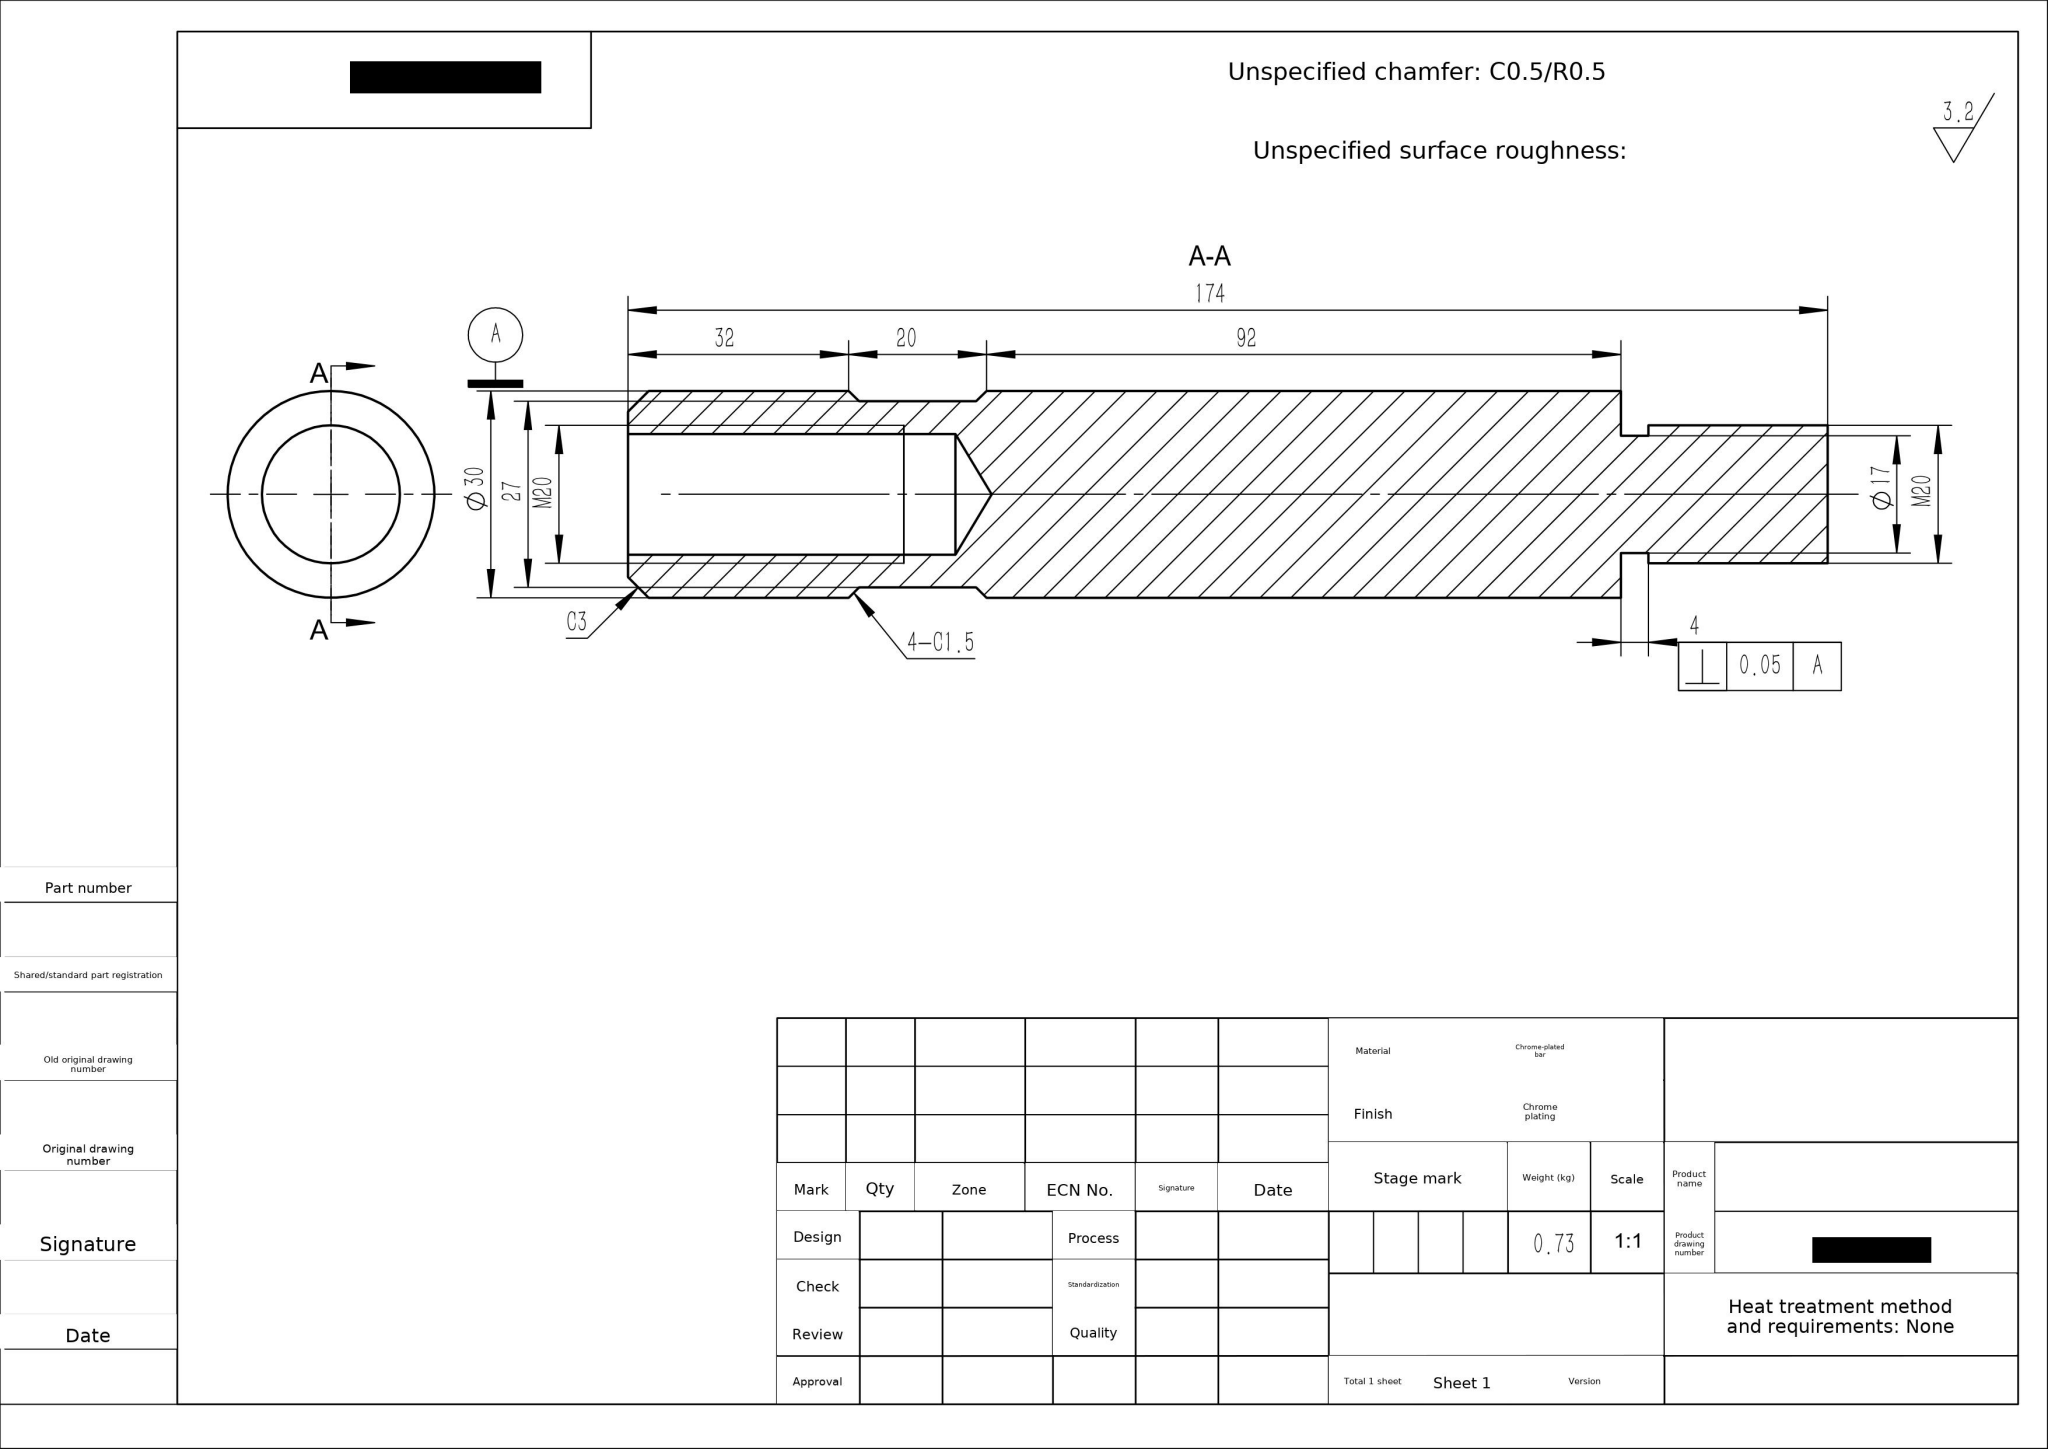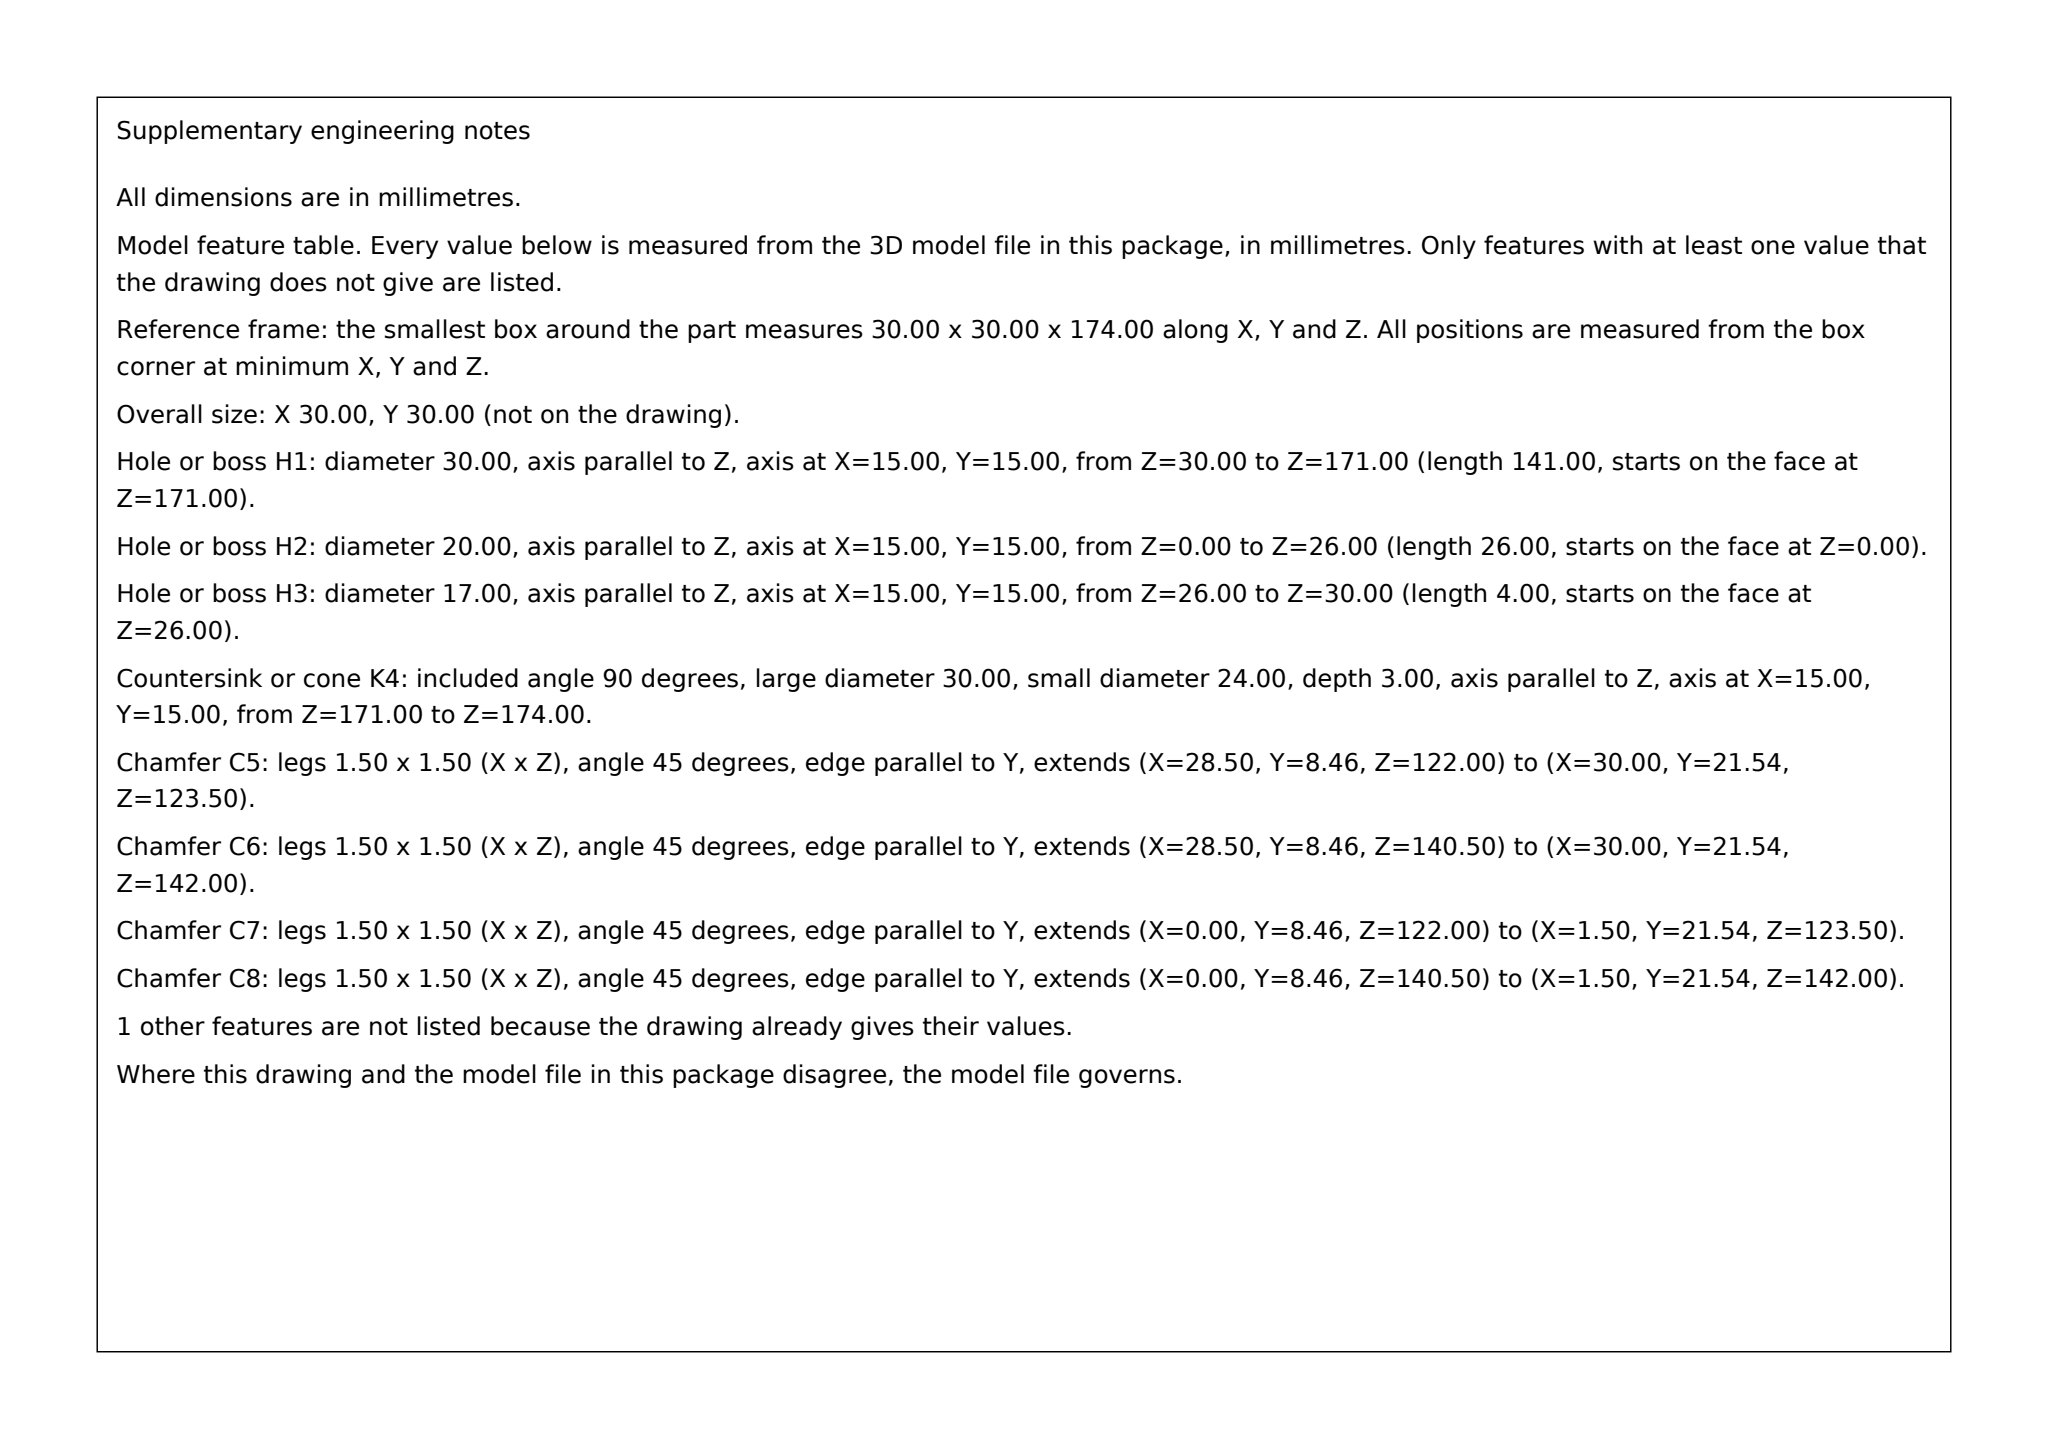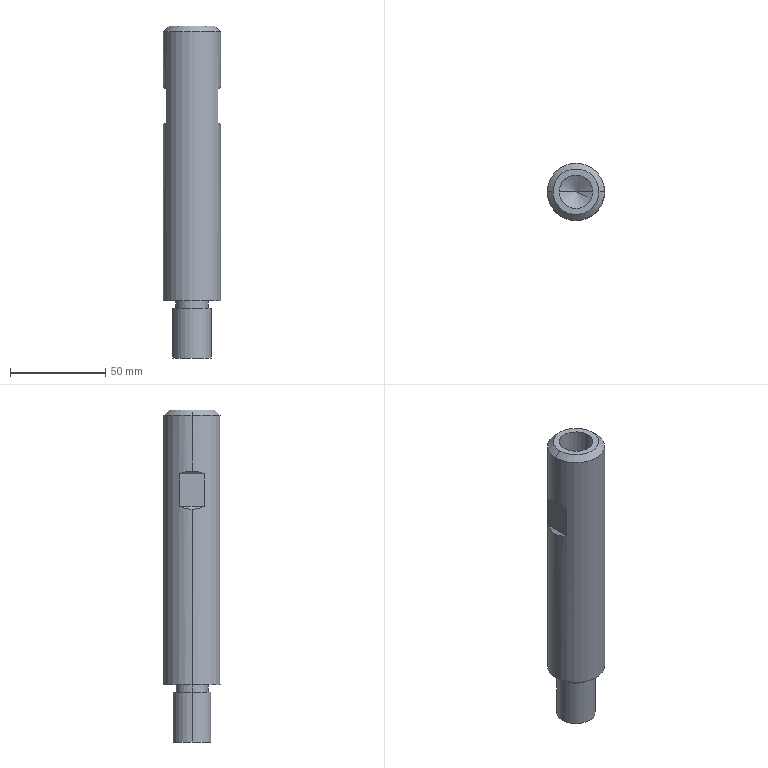Part | SolidWorks | mm | material Chrome-plated bar | 1 solid | 22 faces | box 30 x 30 x 174 mm | volume 98140 mm3 | plane 10 | cylinder 8 | cone 4 | commonest cylinder face diameters 20 x2 17 x2 17.5 x2 30 x2
STEP:
#1=CARTESIAN_POINT('',(12.,0.,174.));
#2=VERTEX_POINT('',#1);
#3=CARTESIAN_POINT('',(-12.,0.,174.));
#4=VERTEX_POINT('',#3);
#5=CARTESIAN_POINT('',(0.,0.,174.));
#6=DIRECTION('',(0.,0.,1.));
#7=DIRECTION('',(1.,0.,0.));
#8=AXIS2_PLACEMENT_3D('',#5,#6,#7);
#9=CIRCLE('',#8,12.);
#10=EDGE_CURVE('',#2,#4,#9,.T.);
#11=ORIENTED_EDGE('',*,*,#10,.F.);
#12=CARTESIAN_POINT('',(15.,0.,171.));
#13=VERTEX_POINT('',#12);
#14=CARTESIAN_POINT('',(12.,0.,174.));
#15=DIRECTION('',(0.7071,0.,-0.7071));
#16=VECTOR('',#15,1000.);
#17=LINE('',#14,#16);
#18=EDGE_CURVE('',#2,#13,#17,.T.);
#19=ORIENTED_EDGE('',*,*,#18,.T.);
#20=CARTESIAN_POINT('',(-15.,0.,171.));
#21=VERTEX_POINT('',#20);
#22=CARTESIAN_POINT('',(0.,0.,171.));
#23=DIRECTION('',(0.,0.,-1.));
#24=DIRECTION('',(1.,0.,0.));
#25=AXIS2_PLACEMENT_3D('',#22,#23,#24);
#26=CIRCLE('',#25,15.);
#27=EDGE_CURVE('',#21,#13,#26,.T.);
#28=ORIENTED_EDGE('',*,*,#27,.F.);
#29=CARTESIAN_POINT('',(-12.,0.,174.));
#30=DIRECTION('',(-0.7071,0.,-0.7071));
#31=VECTOR('',#30,1000.);
#32=LINE('',#29,#31);
#33=EDGE_CURVE('',#4,#21,#32,.T.);
#34=ORIENTED_EDGE('',*,*,#33,.F.);
#35=EDGE_LOOP('',(#11,#19,#28,#34));
#36=FACE_OUTER_BOUND('',#35,.T.);
#37=CARTESIAN_POINT('',(0.,0.,174.));
#38=DIRECTION('',(0.,0.,-1.));
#39=DIRECTION('',(-1.,0.,0.));
#40=AXIS2_PLACEMENT_3D('',#37,#38,#39);
#41=CONICAL_SURFACE('',#40,12.,0.7854);
#42=ADVANCED_FACE('',(#36),#41,.T.);
#43=CARTESIAN_POINT('',(10.,0.,26.));
#44=VERTEX_POINT('',#43);
#45=CARTESIAN_POINT('',(-10.,0.,26.));
#46=VERTEX_POINT('',#45);
#47=CARTESIAN_POINT('',(0.,0.,26.));
#48=DIRECTION('',(0.,0.,1.));
#49=DIRECTION('',(-1.,0.,0.));
#50=AXIS2_PLACEMENT_3D('',#47,#48,#49);
#51=CIRCLE('',#50,10.);
#52=EDGE_CURVE('',#44,#46,#51,.T.);
#53=ORIENTED_EDGE('',*,*,#52,.F.);
#54=CARTESIAN_POINT('',(10.,0.,0.));
#55=VERTEX_POINT('',#54);
#56=CARTESIAN_POINT('',(10.,0.,30.));
#57=DIRECTION('',(0.,0.,-1.));
#58=VECTOR('',#57,1000.);
#59=LINE('',#56,#58);
#60=EDGE_CURVE('',#44,#55,#59,.T.);
#61=ORIENTED_EDGE('',*,*,#60,.T.);
#62=CARTESIAN_POINT('',(-10.,0.,0.));
#63=VERTEX_POINT('',#62);
#64=CARTESIAN_POINT('',(0.,0.,0.));
#65=DIRECTION('',(0.,0.,-1.));
#66=DIRECTION('',(-1.,0.,0.));
#67=AXIS2_PLACEMENT_3D('',#64,#65,#66);
#68=CIRCLE('',#67,10.);
#69=EDGE_CURVE('',#63,#55,#68,.T.);
#70=ORIENTED_EDGE('',*,*,#69,.F.);
#71=CARTESIAN_POINT('',(-10.,0.,30.));
#72=DIRECTION('',(0.,0.,-1.));
#73=VECTOR('',#72,1000.);
#74=LINE('',#71,#73);
#75=EDGE_CURVE('',#46,#63,#74,.T.);
#76=ORIENTED_EDGE('',*,*,#75,.F.);
#77=EDGE_LOOP('',(#53,#61,#70,#76));
#78=FACE_OUTER_BOUND('',#77,.T.);
#79=CARTESIAN_POINT('',(0.,0.,30.));
#80=DIRECTION('',(0.,0.,-1.));
#81=DIRECTION('',(-1.,0.,0.));
#82=AXIS2_PLACEMENT_3D('',#79,#80,#81);
#83=CYLINDRICAL_SURFACE('',#82,10.);
#84=ADVANCED_FACE('',(#78),#83,.T.);
#85=CARTESIAN_POINT('',(-8.5,0.,26.));
#86=VERTEX_POINT('',#85);
#87=CARTESIAN_POINT('',(8.5,0.,26.));
#88=VERTEX_POINT('',#87);
#89=CARTESIAN_POINT('',(0.,0.,26.));
#90=DIRECTION('',(0.,0.,-1.));
#91=DIRECTION('',(-1.,0.,0.));
#92=AXIS2_PLACEMENT_3D('',#89,#90,#91);
#93=CIRCLE('',#92,8.5);
#94=EDGE_CURVE('',#86,#88,#93,.T.);
#95=ORIENTED_EDGE('',*,*,#94,.F.);
#96=CARTESIAN_POINT('',(-8.5,0.,30.));
#97=VERTEX_POINT('',#96);
#98=CARTESIAN_POINT('',(-8.5,0.,26.));
#99=DIRECTION('',(0.,0.,1.));
#100=VECTOR('',#99,1000.);
#101=LINE('',#98,#100);
#102=EDGE_CURVE('',#86,#97,#101,.T.);
#103=ORIENTED_EDGE('',*,*,#102,.T.);
#104=CARTESIAN_POINT('',(8.5,0.,30.));
#105=VERTEX_POINT('',#104);
#106=CARTESIAN_POINT('',(0.,0.,30.));
#107=DIRECTION('',(0.,0.,-1.));
#108=DIRECTION('',(-1.,0.,0.));
#109=AXIS2_PLACEMENT_3D('',#106,#107,#108);
#110=CIRCLE('',#109,8.5);
#111=EDGE_CURVE('',#97,#105,#110,.T.);
#112=ORIENTED_EDGE('',*,*,#111,.T.);
#113=CARTESIAN_POINT('',(8.5,0.,26.));
#114=DIRECTION('',(0.,0.,1.));
#115=VECTOR('',#114,1000.);
#116=LINE('',#113,#115);
#117=EDGE_CURVE('',#88,#105,#116,.T.);
#118=ORIENTED_EDGE('',*,*,#117,.F.);
#119=EDGE_LOOP('',(#95,#103,#112,#118));
#120=FACE_OUTER_BOUND('',#119,.T.);
#121=CARTESIAN_POINT('',(0.,0.,26.));
#122=DIRECTION('',(0.,0.,1.));
#123=DIRECTION('',(1.,0.,0.));
#124=AXIS2_PLACEMENT_3D('',#121,#122,#123);
#125=CYLINDRICAL_SURFACE('',#124,8.5);
#126=ADVANCED_FACE('',(#120),#125,.T.);
#127=CARTESIAN_POINT('',(-8.75,0.,126.5));
#128=VERTEX_POINT('',#127);
#129=CARTESIAN_POINT('',(8.75,0.,126.5));
#130=VERTEX_POINT('',#129);
#131=CARTESIAN_POINT('',(0.,0.,126.5));
#132=DIRECTION('',(0.,0.,1.));
#133=DIRECTION('',(1.,0.,0.));
#134=AXIS2_PLACEMENT_3D('',#131,#132,#133);
#135=CIRCLE('',#134,8.75);
#136=EDGE_CURVE('',#128,#130,#135,.T.);
#137=ORIENTED_EDGE('',*,*,#136,.F.);
#138=CARTESIAN_POINT('',(-8.75,0.,174.));
#139=VERTEX_POINT('',#138);
#140=CARTESIAN_POINT('',(-8.75,0.,174.));
#141=DIRECTION('',(0.,0.,1.));
#142=VECTOR('',#141,1000.);
#143=LINE('',#140,#142);
#144=EDGE_CURVE('',#128,#139,#143,.T.);
#145=ORIENTED_EDGE('',*,*,#144,.T.);
#146=CARTESIAN_POINT('',(8.75,0.,174.));
#147=VERTEX_POINT('',#146);
#148=CARTESIAN_POINT('',(0.,0.,174.));
#149=DIRECTION('',(0.,0.,1.));
#150=DIRECTION('',(1.,0.,0.));
#151=AXIS2_PLACEMENT_3D('',#148,#149,#150);
#152=CIRCLE('',#151,8.75);
#153=EDGE_CURVE('',#139,#147,#152,.T.);
#154=ORIENTED_EDGE('',*,*,#153,.T.);
#155=CARTESIAN_POINT('',(8.75,0.,174.));
#156=DIRECTION('',(0.,0.,1.));
#157=VECTOR('',#156,1000.);
#158=LINE('',#155,#157);
#159=EDGE_CURVE('',#130,#147,#158,.T.);
#160=ORIENTED_EDGE('',*,*,#159,.F.);
#161=EDGE_LOOP('',(#137,#145,#154,#160));
#162=FACE_OUTER_BOUND('',#161,.T.);
#163=CARTESIAN_POINT('',(0.,0.,174.));
#164=DIRECTION('',(0.,0.,1.));
#165=DIRECTION('',(1.,0.,0.));
#166=AXIS2_PLACEMENT_3D('',#163,#164,#165);
#167=CYLINDRICAL_SURFACE('',#166,8.75);
#168=ADVANCED_FACE('',(#162),#167,.F.);
#169=CARTESIAN_POINT('',(-0.,0.,121.242));
#170=VERTEX_POINT('',#169);
#171=CARTESIAN_POINT('',(8.75,0.,126.5));
#172=DIRECTION('',(0.8572,0.,0.515));
#173=VECTOR('',#172,1000.);
#174=LINE('',#171,#173);
#175=EDGE_CURVE('',#170,#130,#174,.T.);
#176=ORIENTED_EDGE('',*,*,#175,.F.);
#177=CARTESIAN_POINT('',(-8.75,0.,126.5));
#178=DIRECTION('',(-0.8572,0.,0.515));
#179=VECTOR('',#178,1000.);
#180=LINE('',#177,#179);
#181=EDGE_CURVE('',#170,#128,#180,.T.);
#182=ORIENTED_EDGE('',*,*,#181,.T.);
#183=ORIENTED_EDGE('',*,*,#136,.T.);
#184=EDGE_LOOP('',(#176,#182,#183));
#185=FACE_OUTER_BOUND('',#184,.T.);
#186=CARTESIAN_POINT('',(0.,0.,126.5));
#187=DIRECTION('',(0.,0.,1.));
#188=DIRECTION('',(1.,0.,0.));
#189=AXIS2_PLACEMENT_3D('',#186,#187,#188);
#190=CONICAL_SURFACE('',#189,8.75,1.03);
#191=ADVANCED_FACE('',(#185),#190,.F.);
#192=ORIENTED_EDGE('',*,*,#27,.T.);
#193=CARTESIAN_POINT('',(15.,0.,142.));
#194=VERTEX_POINT('',#193);
#195=CARTESIAN_POINT('',(15.,0.,174.));
#196=DIRECTION('',(0.,0.,-1.));
#197=VECTOR('',#196,1000.);
#198=LINE('',#195,#197);
#199=EDGE_CURVE('',#13,#194,#198,.T.);
#200=ORIENTED_EDGE('',*,*,#199,.T.);
#201=CARTESIAN_POINT('',(13.5,6.538,140.5));
#202=VERTEX_POINT('',#201);
#203=CARTESIAN_POINT('',(15.,0.,142.));
#204=CARTESIAN_POINT('',(15.,2.274,142.));
#205=CARTESIAN_POINT('',(14.491,4.491,141.491));
#206=CARTESIAN_POINT('',(13.5,6.538,140.5));
#207=(BOUNDED_CURVE()B_SPLINE_CURVE(3,(#203,#204,#205,#206),.UNSPECIFIED.,.F.,.T.)B_SPLINE_CURVE_WITH_KNOTS((4,4),(3.142,3.593),.UNSPECIFIED.)CURVE()GEOMETRIC_REPRESENTATION_ITEM()RATIONAL_B_SPLINE_CURVE((1.,0.9831,0.9831,1.))REPRESENTATION_ITEM(''));
#208=EDGE_CURVE('',#194,#202,#207,.T.);
#209=ORIENTED_EDGE('',*,*,#208,.T.);
#210=CARTESIAN_POINT('',(13.5,6.538,123.5));
#211=VERTEX_POINT('',#210);
#212=CARTESIAN_POINT('',(13.5,6.538,174.));
#213=DIRECTION('',(0.,0.,1.));
#214=VECTOR('',#213,1000.);
#215=LINE('',#212,#214);
#216=EDGE_CURVE('',#211,#202,#215,.T.);
#217=ORIENTED_EDGE('',*,*,#216,.F.);
#218=CARTESIAN_POINT('',(15.,0.,122.));
#219=VERTEX_POINT('',#218);
#220=CARTESIAN_POINT('',(13.5,6.538,123.5));
#221=CARTESIAN_POINT('',(14.491,4.491,122.509));
#222=CARTESIAN_POINT('',(15.,2.274,122.));
#223=CARTESIAN_POINT('',(15.,0.,122.));
#224=(BOUNDED_CURVE()B_SPLINE_CURVE(3,(#220,#221,#222,#223),.UNSPECIFIED.,.F.,.T.)B_SPLINE_CURVE_WITH_KNOTS((4,4),(5.832,6.283),.UNSPECIFIED.)CURVE()GEOMETRIC_REPRESENTATION_ITEM()RATIONAL_B_SPLINE_CURVE((1.,0.9831,0.9831,1.))REPRESENTATION_ITEM(''));
#225=EDGE_CURVE('',#211,#219,#224,.T.);
#226=ORIENTED_EDGE('',*,*,#225,.T.);
#227=CARTESIAN_POINT('',(15.,0.,30.));
#228=VERTEX_POINT('',#227);
#229=CARTESIAN_POINT('',(15.,0.,174.));
#230=DIRECTION('',(0.,0.,-1.));
#231=VECTOR('',#230,1000.);
#232=LINE('',#229,#231);
#233=EDGE_CURVE('',#219,#228,#232,.T.);
#234=ORIENTED_EDGE('',*,*,#233,.T.);
#235=CARTESIAN_POINT('',(-15.,0.,30.));
#236=VERTEX_POINT('',#235);
#237=CARTESIAN_POINT('',(0.,0.,30.));
#238=DIRECTION('',(0.,0.,-1.));
#239=DIRECTION('',(-1.,0.,0.));
#240=AXIS2_PLACEMENT_3D('',#237,#238,#239);
#241=CIRCLE('',#240,15.);
#242=EDGE_CURVE('',#236,#228,#241,.T.);
#243=ORIENTED_EDGE('',*,*,#242,.F.);
#244=CARTESIAN_POINT('',(-15.,0.,122.));
#245=VERTEX_POINT('',#244);
#246=CARTESIAN_POINT('',(-15.,0.,174.));
#247=DIRECTION('',(0.,0.,-1.));
#248=VECTOR('',#247,1000.);
#249=LINE('',#246,#248);
#250=EDGE_CURVE('',#245,#236,#249,.T.);
#251=ORIENTED_EDGE('',*,*,#250,.F.);
#252=CARTESIAN_POINT('',(-13.5,6.538,123.5));
#253=VERTEX_POINT('',#252);
#254=CARTESIAN_POINT('',(-15.,0.,122.));
#255=CARTESIAN_POINT('',(-15.,2.274,122.));
#256=CARTESIAN_POINT('',(-14.491,4.491,122.509));
#257=CARTESIAN_POINT('',(-13.5,6.538,123.5));
#258=(BOUNDED_CURVE()B_SPLINE_CURVE(3,(#254,#255,#256,#257),.UNSPECIFIED.,.F.,.T.)B_SPLINE_CURVE_WITH_KNOTS((4,4),(0.,0.451),.UNSPECIFIED.)CURVE()GEOMETRIC_REPRESENTATION_ITEM()RATIONAL_B_SPLINE_CURVE((1.,0.9831,0.9831,1.))REPRESENTATION_ITEM(''));
#259=EDGE_CURVE('',#245,#253,#258,.T.);
#260=ORIENTED_EDGE('',*,*,#259,.T.);
#261=CARTESIAN_POINT('',(-13.5,6.538,140.5));
#262=VERTEX_POINT('',#261);
#263=CARTESIAN_POINT('',(-13.5,6.538,174.));
#264=DIRECTION('',(0.,0.,-1.));
#265=VECTOR('',#264,1000.);
#266=LINE('',#263,#265);
#267=EDGE_CURVE('',#262,#253,#266,.T.);
#268=ORIENTED_EDGE('',*,*,#267,.F.);
#269=CARTESIAN_POINT('',(-15.,0.,142.));
#270=VERTEX_POINT('',#269);
#271=CARTESIAN_POINT('',(-13.5,6.538,140.5));
#272=CARTESIAN_POINT('',(-14.491,4.491,141.491));
#273=CARTESIAN_POINT('',(-15.,2.274,142.));
#274=CARTESIAN_POINT('',(-15.,0.,142.));
#275=(BOUNDED_CURVE()B_SPLINE_CURVE(3,(#271,#272,#273,#274),.UNSPECIFIED.,.F.,.T.)B_SPLINE_CURVE_WITH_KNOTS((4,4),(2.691,3.142),.UNSPECIFIED.)CURVE()GEOMETRIC_REPRESENTATION_ITEM()RATIONAL_B_SPLINE_CURVE((1.,0.9831,0.9831,1.))REPRESENTATION_ITEM(''));
#276=EDGE_CURVE('',#262,#270,#275,.T.);
#277=ORIENTED_EDGE('',*,*,#276,.T.);
#278=CARTESIAN_POINT('',(-15.,0.,174.));
#279=DIRECTION('',(0.,0.,-1.));
#280=VECTOR('',#279,1000.);
#281=LINE('',#278,#280);
#282=EDGE_CURVE('',#21,#270,#281,.T.);
#283=ORIENTED_EDGE('',*,*,#282,.F.);
#284=EDGE_LOOP('',(#192,#200,#209,#217,#226,#234,#243,#251,#260,#268,#277,#283));
#285=FACE_OUTER_BOUND('',#284,.T.);
#286=CARTESIAN_POINT('',(0.,0.,174.));
#287=DIRECTION('',(0.,0.,-1.));
#288=DIRECTION('',(-1.,0.,0.));
#289=AXIS2_PLACEMENT_3D('',#286,#287,#288);
#290=CYLINDRICAL_SURFACE('',#289,15.);
#291=ADVANCED_FACE('',(#285),#290,.T.);
#292=ORIENTED_EDGE('',*,*,#199,.F.);
#293=CARTESIAN_POINT('',(0.,0.,171.));
#294=DIRECTION('',(0.,0.,-1.));
#295=DIRECTION('',(1.,0.,0.));
#296=AXIS2_PLACEMENT_3D('',#293,#294,#295);
#297=CIRCLE('',#296,15.);
#298=EDGE_CURVE('',#13,#21,#297,.T.);
#299=ORIENTED_EDGE('',*,*,#298,.T.);
#300=ORIENTED_EDGE('',*,*,#282,.T.);
#301=CARTESIAN_POINT('',(-13.5,-6.538,140.5));
#302=VERTEX_POINT('',#301);
#303=CARTESIAN_POINT('',(-15.,0.,142.));
#304=CARTESIAN_POINT('',(-15.,-2.274,142.));
#305=CARTESIAN_POINT('',(-14.491,-4.491,141.491));
#306=CARTESIAN_POINT('',(-13.5,-6.538,140.5));
#307=(BOUNDED_CURVE()B_SPLINE_CURVE(3,(#303,#304,#305,#306),.UNSPECIFIED.,.F.,.T.)B_SPLINE_CURVE_WITH_KNOTS((4,4),(3.142,3.593),.UNSPECIFIED.)CURVE()GEOMETRIC_REPRESENTATION_ITEM()RATIONAL_B_SPLINE_CURVE((1.,0.9831,0.9831,1.))REPRESENTATION_ITEM(''));
#308=EDGE_CURVE('',#270,#302,#307,.T.);
#309=ORIENTED_EDGE('',*,*,#308,.T.);
#310=CARTESIAN_POINT('',(-13.5,-6.538,123.5));
#311=VERTEX_POINT('',#310);
#312=CARTESIAN_POINT('',(-13.5,-6.538,174.));
#313=DIRECTION('',(0.,0.,1.));
#314=VECTOR('',#313,1000.);
#315=LINE('',#312,#314);
#316=EDGE_CURVE('',#311,#302,#315,.T.);
#317=ORIENTED_EDGE('',*,*,#316,.F.);
#318=CARTESIAN_POINT('',(-13.5,-6.538,123.5));
#319=CARTESIAN_POINT('',(-14.491,-4.491,122.509));
#320=CARTESIAN_POINT('',(-15.,-2.274,122.));
#321=CARTESIAN_POINT('',(-15.,0.,122.));
#322=(BOUNDED_CURVE()B_SPLINE_CURVE(3,(#318,#319,#320,#321),.UNSPECIFIED.,.F.,.T.)B_SPLINE_CURVE_WITH_KNOTS((4,4),(5.832,6.283),.UNSPECIFIED.)CURVE()GEOMETRIC_REPRESENTATION_ITEM()RATIONAL_B_SPLINE_CURVE((1.,0.9831,0.9831,1.))REPRESENTATION_ITEM(''));
#323=EDGE_CURVE('',#311,#245,#322,.T.);
#324=ORIENTED_EDGE('',*,*,#323,.T.);
#325=ORIENTED_EDGE('',*,*,#250,.T.);
#326=CARTESIAN_POINT('',(0.,0.,30.));
#327=DIRECTION('',(0.,0.,-1.));
#328=DIRECTION('',(-1.,0.,0.));
#329=AXIS2_PLACEMENT_3D('',#326,#327,#328);
#330=CIRCLE('',#329,15.);
#331=EDGE_CURVE('',#228,#236,#330,.T.);
#332=ORIENTED_EDGE('',*,*,#331,.F.);
#333=ORIENTED_EDGE('',*,*,#233,.F.);
#334=CARTESIAN_POINT('',(13.5,-6.538,123.5));
#335=VERTEX_POINT('',#334);
#336=CARTESIAN_POINT('',(15.,0.,122.));
#337=CARTESIAN_POINT('',(15.,-2.274,122.));
#338=CARTESIAN_POINT('',(14.491,-4.491,122.509));
#339=CARTESIAN_POINT('',(13.5,-6.538,123.5));
#340=(BOUNDED_CURVE()B_SPLINE_CURVE(3,(#336,#337,#338,#339),.UNSPECIFIED.,.F.,.T.)B_SPLINE_CURVE_WITH_KNOTS((4,4),(0.,0.451),.UNSPECIFIED.)CURVE()GEOMETRIC_REPRESENTATION_ITEM()RATIONAL_B_SPLINE_CURVE((1.,0.9831,0.9831,1.))REPRESENTATION_ITEM(''));
#341=EDGE_CURVE('',#219,#335,#340,.T.);
#342=ORIENTED_EDGE('',*,*,#341,.T.);
#343=CARTESIAN_POINT('',(13.5,-6.538,140.5));
#344=VERTEX_POINT('',#343);
#345=CARTESIAN_POINT('',(13.5,-6.538,174.));
#346=DIRECTION('',(0.,0.,-1.));
#347=VECTOR('',#346,1000.);
#348=LINE('',#345,#347);
#349=EDGE_CURVE('',#344,#335,#348,.T.);
#350=ORIENTED_EDGE('',*,*,#349,.F.);
#351=CARTESIAN_POINT('',(13.5,-6.538,140.5));
#352=CARTESIAN_POINT('',(14.491,-4.491,141.491));
#353=CARTESIAN_POINT('',(15.,-2.274,142.));
#354=CARTESIAN_POINT('',(15.,0.,142.));
#355=(BOUNDED_CURVE()B_SPLINE_CURVE(3,(#351,#352,#353,#354),.UNSPECIFIED.,.F.,.T.)B_SPLINE_CURVE_WITH_KNOTS((4,4),(2.691,3.142),.UNSPECIFIED.)CURVE()GEOMETRIC_REPRESENTATION_ITEM()RATIONAL_B_SPLINE_CURVE((1.,0.9831,0.9831,1.))REPRESENTATION_ITEM(''));
#356=EDGE_CURVE('',#344,#194,#355,.T.);
#357=ORIENTED_EDGE('',*,*,#356,.T.);
#358=EDGE_LOOP('',(#292,#299,#300,#309,#317,#324,#325,#332,#333,#342,#350,#357));
#359=FACE_OUTER_BOUND('',#358,.T.);
#360=CARTESIAN_POINT('',(0.,0.,174.));
#361=DIRECTION('',(0.,0.,-1.));
#362=DIRECTION('',(-1.,0.,0.));
#363=AXIS2_PLACEMENT_3D('',#360,#361,#362);
#364=CYLINDRICAL_SURFACE('',#363,15.);
#365=ADVANCED_FACE('',(#359),#364,.T.);
#366=CARTESIAN_POINT('',(0.,0.,174.));
#367=DIRECTION('',(0.,0.,1.));
#368=DIRECTION('',(1.,0.,0.));
#369=AXIS2_PLACEMENT_3D('',#366,#367,#368);
#370=CIRCLE('',#369,12.);
#371=EDGE_CURVE('',#4,#2,#370,.T.);
#372=ORIENTED_EDGE('',*,*,#371,.T.);
#373=ORIENTED_EDGE('',*,*,#10,.T.);
#374=EDGE_LOOP('',(#372,#373));
#375=FACE_OUTER_BOUND('',#374,.T.);
#376=CARTESIAN_POINT('',(0.,0.,174.));
#377=DIRECTION('',(0.,0.,1.));
#378=DIRECTION('',(1.,0.,0.));
#379=AXIS2_PLACEMENT_3D('',#376,#377,#378);
#380=CIRCLE('',#379,8.75);
#381=EDGE_CURVE('',#147,#139,#380,.T.);
#382=ORIENTED_EDGE('',*,*,#381,.F.);
#383=ORIENTED_EDGE('',*,*,#153,.F.);
#384=EDGE_LOOP('',(#382,#383));
#385=FACE_BOUND('',#384,.T.);
#386=CARTESIAN_POINT('',(0.,0.,174.));
#387=DIRECTION('',(0.,0.,1.));
#388=DIRECTION('',(1.,0.,0.));
#389=AXIS2_PLACEMENT_3D('',#386,#387,#388);
#390=PLANE('',#389);
#391=ADVANCED_FACE('',(#375,#385),#390,.T.);
#392=ORIENTED_EDGE('',*,*,#181,.F.);
#393=ORIENTED_EDGE('',*,*,#175,.T.);
#394=CARTESIAN_POINT('',(0.,0.,126.5));
#395=DIRECTION('',(0.,0.,1.));
#396=DIRECTION('',(1.,0.,0.));
#397=AXIS2_PLACEMENT_3D('',#394,#395,#396);
#398=CIRCLE('',#397,8.75);
#399=EDGE_CURVE('',#130,#128,#398,.T.);
#400=ORIENTED_EDGE('',*,*,#399,.T.);
#401=EDGE_LOOP('',(#392,#393,#400));
#402=FACE_OUTER_BOUND('',#401,.T.);
#403=CARTESIAN_POINT('',(0.,0.,126.5));
#404=DIRECTION('',(0.,0.,1.));
#405=DIRECTION('',(1.,0.,0.));
#406=AXIS2_PLACEMENT_3D('',#403,#404,#405);
#407=CONICAL_SURFACE('',#406,8.75,1.03);
#408=ADVANCED_FACE('',(#402),#407,.F.);
#409=ORIENTED_EDGE('',*,*,#144,.F.);
#410=ORIENTED_EDGE('',*,*,#399,.F.);
#411=ORIENTED_EDGE('',*,*,#159,.T.);
#412=ORIENTED_EDGE('',*,*,#381,.T.);
#413=EDGE_LOOP('',(#409,#410,#411,#412));
#414=FACE_OUTER_BOUND('',#413,.T.);
#415=CARTESIAN_POINT('',(0.,0.,174.));
#416=DIRECTION('',(0.,0.,1.));
#417=DIRECTION('',(1.,0.,0.));
#418=AXIS2_PLACEMENT_3D('',#415,#416,#417);
#419=CYLINDRICAL_SURFACE('',#418,8.75);
#420=ADVANCED_FACE('',(#414),#419,.F.);
#421=ORIENTED_EDGE('',*,*,#242,.T.);
#422=ORIENTED_EDGE('',*,*,#331,.T.);
#423=EDGE_LOOP('',(#421,#422));
#424=FACE_OUTER_BOUND('',#423,.T.);
#425=CARTESIAN_POINT('',(0.,0.,30.));
#426=DIRECTION('',(0.,0.,-1.));
#427=DIRECTION('',(-1.,0.,0.));
#428=AXIS2_PLACEMENT_3D('',#425,#426,#427);
#429=CIRCLE('',#428,8.5);
#430=EDGE_CURVE('',#105,#97,#429,.T.);
#431=ORIENTED_EDGE('',*,*,#430,.F.);
#432=ORIENTED_EDGE('',*,*,#111,.F.);
#433=EDGE_LOOP('',(#431,#432));
#434=FACE_BOUND('',#433,.T.);
#435=CARTESIAN_POINT('',(0.,0.,30.));
#436=DIRECTION('',(0.,0.,-1.));
#437=DIRECTION('',(-1.,0.,0.));
#438=AXIS2_PLACEMENT_3D('',#435,#436,#437);
#439=PLANE('',#438);
#440=ADVANCED_FACE('',(#424,#434),#439,.T.);
#441=CARTESIAN_POINT('',(0.,0.,26.));
#442=DIRECTION('',(0.,0.,1.));
#443=DIRECTION('',(-1.,0.,0.));
#444=AXIS2_PLACEMENT_3D('',#441,#442,#443);
#445=CIRCLE('',#444,10.);
#446=EDGE_CURVE('',#46,#44,#445,.T.);
#447=ORIENTED_EDGE('',*,*,#446,.T.);
#448=ORIENTED_EDGE('',*,*,#52,.T.);
#449=EDGE_LOOP('',(#447,#448));
#450=FACE_OUTER_BOUND('',#449,.T.);
#451=CARTESIAN_POINT('',(0.,0.,26.));
#452=DIRECTION('',(0.,0.,-1.));
#453=DIRECTION('',(-1.,0.,0.));
#454=AXIS2_PLACEMENT_3D('',#451,#452,#453);
#455=CIRCLE('',#454,8.5);
#456=EDGE_CURVE('',#88,#86,#455,.T.);
#457=ORIENTED_EDGE('',*,*,#456,.T.);
#458=ORIENTED_EDGE('',*,*,#94,.T.);
#459=EDGE_LOOP('',(#457,#458));
#460=FACE_BOUND('',#459,.T.);
#461=CARTESIAN_POINT('',(0.,0.,26.));
#462=DIRECTION('',(0.,0.,-1.));
#463=DIRECTION('',(-1.,0.,0.));
#464=AXIS2_PLACEMENT_3D('',#461,#462,#463);
#465=PLANE('',#464);
#466=ADVANCED_FACE('',(#450,#460),#465,.F.);
#467=ORIENTED_EDGE('',*,*,#102,.F.);
#468=ORIENTED_EDGE('',*,*,#456,.F.);
#469=ORIENTED_EDGE('',*,*,#117,.T.);
#470=ORIENTED_EDGE('',*,*,#430,.T.);
#471=EDGE_LOOP('',(#467,#468,#469,#470));
#472=FACE_OUTER_BOUND('',#471,.T.);
#473=CARTESIAN_POINT('',(0.,0.,26.));
#474=DIRECTION('',(0.,0.,1.));
#475=DIRECTION('',(1.,0.,0.));
#476=AXIS2_PLACEMENT_3D('',#473,#474,#475);
#477=CYLINDRICAL_SURFACE('',#476,8.5);
#478=ADVANCED_FACE('',(#472),#477,.T.);
#479=ORIENTED_EDGE('',*,*,#69,.T.);
#480=CARTESIAN_POINT('',(0.,0.,0.));
#481=DIRECTION('',(0.,0.,-1.));
#482=DIRECTION('',(-1.,0.,0.));
#483=AXIS2_PLACEMENT_3D('',#480,#481,#482);
#484=CIRCLE('',#483,10.);
#485=EDGE_CURVE('',#55,#63,#484,.T.);
#486=ORIENTED_EDGE('',*,*,#485,.T.);
#487=EDGE_LOOP('',(#479,#486));
#488=FACE_OUTER_BOUND('',#487,.T.);
#489=CARTESIAN_POINT('',(0.,0.,0.));
#490=DIRECTION('',(0.,0.,1.));
#491=DIRECTION('',(1.,0.,0.));
#492=AXIS2_PLACEMENT_3D('',#489,#490,#491);
#493=PLANE('',#492);
#494=ADVANCED_FACE('',(#488),#493,.F.);
#495=ORIENTED_EDGE('',*,*,#60,.F.);
#496=ORIENTED_EDGE('',*,*,#446,.F.);
#497=ORIENTED_EDGE('',*,*,#75,.T.);
#498=ORIENTED_EDGE('',*,*,#485,.F.);
#499=EDGE_LOOP('',(#495,#496,#497,#498));
#500=FACE_OUTER_BOUND('',#499,.T.);
#501=CARTESIAN_POINT('',(0.,0.,30.));
#502=DIRECTION('',(0.,0.,-1.));
#503=DIRECTION('',(-1.,0.,0.));
#504=AXIS2_PLACEMENT_3D('',#501,#502,#503);
#505=CYLINDRICAL_SURFACE('',#504,10.);
#506=ADVANCED_FACE('',(#500),#505,.T.);
#507=ORIENTED_EDGE('',*,*,#267,.T.);
#508=CARTESIAN_POINT('',(-13.5,-6.538,123.5));
#509=DIRECTION('',(0.,-1.,0.));
#510=VECTOR('',#509,1000.);
#511=LINE('',#508,#510);
#512=EDGE_CURVE('',#253,#311,#511,.T.);
#513=ORIENTED_EDGE('',*,*,#512,.T.);
#514=ORIENTED_EDGE('',*,*,#316,.T.);
#515=CARTESIAN_POINT('',(-13.5,25.915,140.5));
#516=DIRECTION('',(-0.,1.,0.));
#517=VECTOR('',#516,1000.);
#518=LINE('',#515,#517);
#519=EDGE_CURVE('',#302,#262,#518,.T.);
#520=ORIENTED_EDGE('',*,*,#519,.T.);
#521=EDGE_LOOP('',(#507,#513,#514,#520));
#522=FACE_OUTER_BOUND('',#521,.T.);
#523=CARTESIAN_POINT('',(-13.5,25.915,122.));
#524=DIRECTION('',(-1.,-0.,0.));
#525=DIRECTION('',(0.,-1.,0.));
#526=AXIS2_PLACEMENT_3D('',#523,#524,#525);
#527=PLANE('',#526);
#528=ADVANCED_FACE('',(#522),#527,.T.);
#529=ORIENTED_EDGE('',*,*,#349,.T.);
#530=CARTESIAN_POINT('',(13.5,6.538,123.5));
#531=DIRECTION('',(-0.,1.,0.));
#532=VECTOR('',#531,1000.);
#533=LINE('',#530,#532);
#534=EDGE_CURVE('',#335,#211,#533,.T.);
#535=ORIENTED_EDGE('',*,*,#534,.T.);
#536=ORIENTED_EDGE('',*,*,#216,.T.);
#537=CARTESIAN_POINT('',(13.5,25.915,140.5));
#538=DIRECTION('',(0.,-1.,0.));
#539=VECTOR('',#538,1000.);
#540=LINE('',#537,#539);
#541=EDGE_CURVE('',#202,#344,#540,.T.);
#542=ORIENTED_EDGE('',*,*,#541,.T.);
#543=EDGE_LOOP('',(#529,#535,#536,#542));
#544=FACE_OUTER_BOUND('',#543,.T.);
#545=CARTESIAN_POINT('',(13.5,25.915,122.));
#546=DIRECTION('',(1.,0.,0.));
#547=DIRECTION('',(-0.,1.,0.));
#548=AXIS2_PLACEMENT_3D('',#545,#546,#547);
#549=PLANE('',#548);
#550=ADVANCED_FACE('',(#544),#549,.T.);
#551=ORIENTED_EDGE('',*,*,#534,.F.);
#552=ORIENTED_EDGE('',*,*,#341,.F.);
#553=ORIENTED_EDGE('',*,*,#225,.F.);
#554=EDGE_LOOP('',(#551,#552,#553));
#555=FACE_OUTER_BOUND('',#554,.T.);
#556=CARTESIAN_POINT('',(13.5,25.915,123.5));
#557=DIRECTION('',(0.7071,0.,0.7071));
#558=DIRECTION('',(0.,-1.,0.));
#559=AXIS2_PLACEMENT_3D('',#556,#557,#558);
#560=PLANE('',#559);
#561=ADVANCED_FACE('',(#555),#560,.T.);
#562=ORIENTED_EDGE('',*,*,#356,.F.);
#563=ORIENTED_EDGE('',*,*,#541,.F.);
#564=ORIENTED_EDGE('',*,*,#208,.F.);
#565=EDGE_LOOP('',(#562,#563,#564));
#566=FACE_OUTER_BOUND('',#565,.T.);
#567=CARTESIAN_POINT('',(15.,0.,142.));
#568=DIRECTION('',(-0.7071,-0.,0.7071));
#569=DIRECTION('',(-0.,1.,0.));
#570=AXIS2_PLACEMENT_3D('',#567,#568,#569);
#571=PLANE('',#570);
#572=ADVANCED_FACE('',(#566),#571,.F.);
#573=ORIENTED_EDGE('',*,*,#512,.F.);
#574=ORIENTED_EDGE('',*,*,#259,.F.);
#575=ORIENTED_EDGE('',*,*,#323,.F.);
#576=EDGE_LOOP('',(#573,#574,#575));
#577=FACE_OUTER_BOUND('',#576,.T.);
#578=CARTESIAN_POINT('',(-13.5,25.915,123.5));
#579=DIRECTION('',(-0.7071,-0.,0.7071));
#580=DIRECTION('',(-0.,1.,0.));
#581=AXIS2_PLACEMENT_3D('',#578,#579,#580);
#582=PLANE('',#581);
#583=ADVANCED_FACE('',(#577),#582,.T.);
#584=ORIENTED_EDGE('',*,*,#276,.F.);
#585=ORIENTED_EDGE('',*,*,#519,.F.);
#586=ORIENTED_EDGE('',*,*,#308,.F.);
#587=EDGE_LOOP('',(#584,#585,#586));
#588=FACE_OUTER_BOUND('',#587,.T.);
#589=CARTESIAN_POINT('',(-15.,-0.,142.));
#590=DIRECTION('',(0.7071,0.,0.7071));
#591=DIRECTION('',(0.,-1.,0.));
#592=AXIS2_PLACEMENT_3D('',#589,#590,#591);
#593=PLANE('',#592);
#594=ADVANCED_FACE('',(#588),#593,.F.);
#595=ORIENTED_EDGE('',*,*,#18,.F.);
#596=ORIENTED_EDGE('',*,*,#371,.F.);
#597=ORIENTED_EDGE('',*,*,#33,.T.);
#598=ORIENTED_EDGE('',*,*,#298,.F.);
#599=EDGE_LOOP('',(#595,#596,#597,#598));
#600=FACE_OUTER_BOUND('',#599,.T.);
#601=CARTESIAN_POINT('',(0.,0.,174.));
#602=DIRECTION('',(0.,0.,-1.));
#603=DIRECTION('',(-1.,0.,0.));
#604=AXIS2_PLACEMENT_3D('',#601,#602,#603);
#605=CONICAL_SURFACE('',#604,12.,0.7854);
#606=ADVANCED_FACE('',(#600),#605,.T.);
#607=CLOSED_SHELL('',(#42,#84,#126,#168,#191,#291,#365,#391,#408,#420,#440,#466,#478,#494,#506,#528,#550,#561,#572,#583,#594,#606));
#608=MANIFOLD_SOLID_BREP('',#607);
#609=CARTESIAN_POINT('',(0.,0.,0.));
#610=DIRECTION('',(0.,0.,1.));
#611=DIRECTION('',(1.,0.,0.));
#612=AXIS2_PLACEMENT_3D('',#609,#610,#611);
#613=(LENGTH_UNIT()NAMED_UNIT(*)SI_UNIT(.MILLI.,.METRE.));
#614=UNCERTAINTY_MEASURE_WITH_UNIT(LENGTH_MEASURE(0.00001),#613,'','');
#615=(NAMED_UNIT(*)PLANE_ANGLE_UNIT()SI_UNIT($,.RADIAN.));
#616=(NAMED_UNIT(*)SI_UNIT($,.STERADIAN.)SOLID_ANGLE_UNIT());
#617=(GEOMETRIC_REPRESENTATION_CONTEXT(3)GLOBAL_UNCERTAINTY_ASSIGNED_CONTEXT((#614))GLOBAL_UNIT_ASSIGNED_CONTEXT((#613,#615,#616))REPRESENTATION_CONTEXT('',''));
#618=ADVANCED_BREP_SHAPE_REPRESENTATION('',(#608,#612),#617);